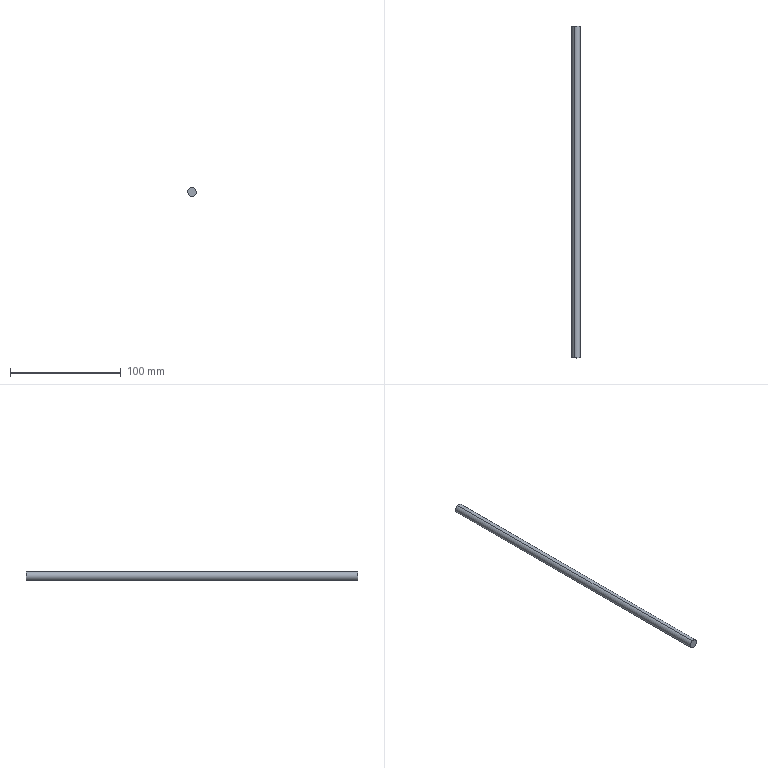Component | SolidWorks | LiftingRod-2 | 1 solid | 4 faces | box 8 x 300 x 8 mm | volume 15080 mm3 | cylinder 2 | plane 2 | commonest cylinder face diameters 8 x2
build123d program:
from build123d import *

# Parameters (mm, degrees)
SKETCH1_R           = 4
BOSS_EXTRUDE1_DEPTH = 300


with BuildPart() as part:
    # Sketch1 → Boss-Extrude1 (new body)
    with BuildSketch(Plane(origin=(0, 0, 0), x_dir=(1, 0, 0), z_dir=(0, 1, 0))):
        with Locations(Location((0, 0, 0), (0, 0, 270))):
            Circle(SKETCH1_R)
    extrude(amount=BOSS_EXTRUDE1_DEPTH)


solid = part.part

# Placed as in the assembly
solid = solid.moved(Location((-88.775, 496.583, 608.366), (0, 0, 0)))
STEP:
#1=COLOUR_RGB('',0.7922,0.8196,0.9333);
#2=FILL_AREA_STYLE_COLOUR('',#1);
#3=FILL_AREA_STYLE('',(#2));
#4=SURFACE_STYLE_FILL_AREA(#3);
#5=SURFACE_SIDE_STYLE('',(#4));
#6=SURFACE_STYLE_USAGE(.BOTH.,#5);
#7=PRESENTATION_STYLE_ASSIGNMENT((#6));
#8=CARTESIAN_POINT('',(-3.548,31.362,24.1));
#9=VERTEX_POINT('',#8);
#10=CARTESIAN_POINT('',(-3.442,31.362,23.803));
#11=VERTEX_POINT('',#10);
#12=CARTESIAN_POINT('',(-3.495,31.362,23.951));
#13=DIRECTION('',(0.,1.,-0.));
#14=DIRECTION('',(-0.3372,0.,0.9415));
#15=AXIS2_PLACEMENT_3D('',#12,#13,#14);
#16=CIRCLE('',#15,0.1575);
#17=EDGE_CURVE('',#9,#11,#16,.T.);
#18=ORIENTED_EDGE('',*,*,#17,.F.);
#19=CARTESIAN_POINT('',(-3.548,19.551,24.1));
#20=VERTEX_POINT('',#19);
#21=CARTESIAN_POINT('',(-3.548,31.362,24.1));
#22=DIRECTION('',(-0.,-1.,0.));
#23=VECTOR('',#22,39.37);
#24=LINE('',#21,#23);
#25=EDGE_CURVE('',#9,#20,#24,.T.);
#26=ORIENTED_EDGE('',*,*,#25,.T.);
#27=CARTESIAN_POINT('',(-3.442,19.551,23.803));
#28=VERTEX_POINT('',#27);
#29=CARTESIAN_POINT('',(-3.495,19.551,23.951));
#30=DIRECTION('',(0.,1.,-0.));
#31=DIRECTION('',(-0.3372,0.,0.9415));
#32=AXIS2_PLACEMENT_3D('',#29,#30,#31);
#33=CIRCLE('',#32,0.1575);
#34=EDGE_CURVE('',#20,#28,#33,.T.);
#35=ORIENTED_EDGE('',*,*,#34,.T.);
#36=CARTESIAN_POINT('',(-3.442,31.362,23.803));
#37=DIRECTION('',(-0.,-1.,0.));
#38=VECTOR('',#37,39.37);
#39=LINE('',#36,#38);
#40=EDGE_CURVE('',#11,#28,#39,.T.);
#41=ORIENTED_EDGE('',*,*,#40,.F.);
#42=EDGE_LOOP('',(#18,#26,#35,#41));
#43=FACE_OUTER_BOUND('',#42,.T.);
#44=CARTESIAN_POINT('',(-3.495,31.362,23.951));
#45=DIRECTION('',(-0.,-1.,0.));
#46=DIRECTION('',(0.3372,0.,-0.9415));
#47=AXIS2_PLACEMENT_3D('',#44,#45,#46);
#48=CYLINDRICAL_SURFACE('',#47,0.1575);
#49=ADVANCED_FACE('',(#43),#48,.T.);
#50=ORIENTED_EDGE('',*,*,#25,.F.);
#51=CARTESIAN_POINT('',(-3.495,31.362,23.951));
#52=DIRECTION('',(0.,1.,-0.));
#53=DIRECTION('',(-0.3372,0.,0.9415));
#54=AXIS2_PLACEMENT_3D('',#51,#52,#53);
#55=CIRCLE('',#54,0.1575);
#56=EDGE_CURVE('',#11,#9,#55,.T.);
#57=ORIENTED_EDGE('',*,*,#56,.F.);
#58=ORIENTED_EDGE('',*,*,#40,.T.);
#59=CARTESIAN_POINT('',(-3.495,19.551,23.951));
#60=DIRECTION('',(0.,1.,-0.));
#61=DIRECTION('',(-0.3372,0.,0.9415));
#62=AXIS2_PLACEMENT_3D('',#59,#60,#61);
#63=CIRCLE('',#62,0.1575);
#64=EDGE_CURVE('',#28,#20,#63,.T.);
#65=ORIENTED_EDGE('',*,*,#64,.T.);
#66=EDGE_LOOP('',(#50,#57,#58,#65));
#67=FACE_OUTER_BOUND('',#66,.T.);
#68=CARTESIAN_POINT('',(-3.495,31.362,23.951));
#69=DIRECTION('',(-0.,-1.,0.));
#70=DIRECTION('',(0.3372,0.,-0.9415));
#71=AXIS2_PLACEMENT_3D('',#68,#69,#70);
#72=CYLINDRICAL_SURFACE('',#71,0.1575);
#73=ADVANCED_FACE('',(#67),#72,.T.);
#74=ORIENTED_EDGE('',*,*,#56,.T.);
#75=ORIENTED_EDGE('',*,*,#17,.T.);
#76=EDGE_LOOP('',(#74,#75));
#77=FACE_OUTER_BOUND('',#76,.T.);
#78=CARTESIAN_POINT('',(-3.495,31.362,23.951));
#79=DIRECTION('',(0.,1.,-0.));
#80=DIRECTION('',(-0.3372,0.,0.9415));
#81=AXIS2_PLACEMENT_3D('',#78,#79,#80);
#82=PLANE('',#81);
#83=ADVANCED_FACE('',(#77),#82,.T.);
#84=ORIENTED_EDGE('',*,*,#64,.F.);
#85=ORIENTED_EDGE('',*,*,#34,.F.);
#86=EDGE_LOOP('',(#84,#85));
#87=FACE_OUTER_BOUND('',#86,.T.);
#88=CARTESIAN_POINT('',(-3.495,19.551,23.951));
#89=DIRECTION('',(0.,1.,-0.));
#90=DIRECTION('',(-0.3372,0.,0.9415));
#91=AXIS2_PLACEMENT_3D('',#88,#89,#90);
#92=PLANE('',#91);
#93=ADVANCED_FACE('',(#87),#92,.F.);
#94=CLOSED_SHELL('',(#49,#73,#83,#93));
#95=MANIFOLD_SOLID_BREP('',#94);
#96=STYLED_ITEM('',(#7),#95);
#97=(LENGTH_UNIT()NAMED_UNIT(*)SI_UNIT($,.METRE.));
#98=LENGTH_MEASURE_WITH_UNIT(LENGTH_MEASURE(0.0254),#97);
#99=DIMENSIONAL_EXPONENTS(1.,0.,0.,0.,0.,0.,0.);
#100=(CONVERSION_BASED_UNIT('',#98)LENGTH_UNIT()NAMED_UNIT(#99));
#101=UNCERTAINTY_MEASURE_WITH_UNIT(LENGTH_MEASURE(0.00001),#100,'','');
#102=(NAMED_UNIT(*)PLANE_ANGLE_UNIT()SI_UNIT($,.RADIAN.));
#103=(NAMED_UNIT(*)SI_UNIT($,.STERADIAN.)SOLID_ANGLE_UNIT());
#104=(GEOMETRIC_REPRESENTATION_CONTEXT(3)GLOBAL_UNCERTAINTY_ASSIGNED_CONTEXT((#101))GLOBAL_UNIT_ASSIGNED_CONTEXT((#100,#102,#103))REPRESENTATION_CONTEXT('',''));
#105=MECHANICAL_DESIGN_GEOMETRIC_PRESENTATION_REPRESENTATION('',(#96),#104);
#106=PRESENTATION_LAYER_ASSIGNMENT('','',(#96));
#107=CARTESIAN_POINT('',(0.,0.,0.));
#108=DIRECTION('',(0.,0.,1.));
#109=DIRECTION('',(1.,0.,0.));
#110=AXIS2_PLACEMENT_3D('',#107,#108,#109);
#111=(LENGTH_UNIT()NAMED_UNIT(*)SI_UNIT($,.METRE.));
#112=LENGTH_MEASURE_WITH_UNIT(LENGTH_MEASURE(0.0254),#111);
#113=DIMENSIONAL_EXPONENTS(1.,0.,0.,0.,0.,0.,0.);
#114=(CONVERSION_BASED_UNIT('',#112)LENGTH_UNIT()NAMED_UNIT(#113));
#115=UNCERTAINTY_MEASURE_WITH_UNIT(LENGTH_MEASURE(0.00001),#114,'','');
#116=(NAMED_UNIT(*)PLANE_ANGLE_UNIT()SI_UNIT($,.RADIAN.));
#117=(NAMED_UNIT(*)SI_UNIT($,.STERADIAN.)SOLID_ANGLE_UNIT());
#118=(GEOMETRIC_REPRESENTATION_CONTEXT(3)GLOBAL_UNCERTAINTY_ASSIGNED_CONTEXT((#115))GLOBAL_UNIT_ASSIGNED_CONTEXT((#114,#116,#117))REPRESENTATION_CONTEXT('',''));
#119=ADVANCED_BREP_SHAPE_REPRESENTATION('',(#95,#110),#118);